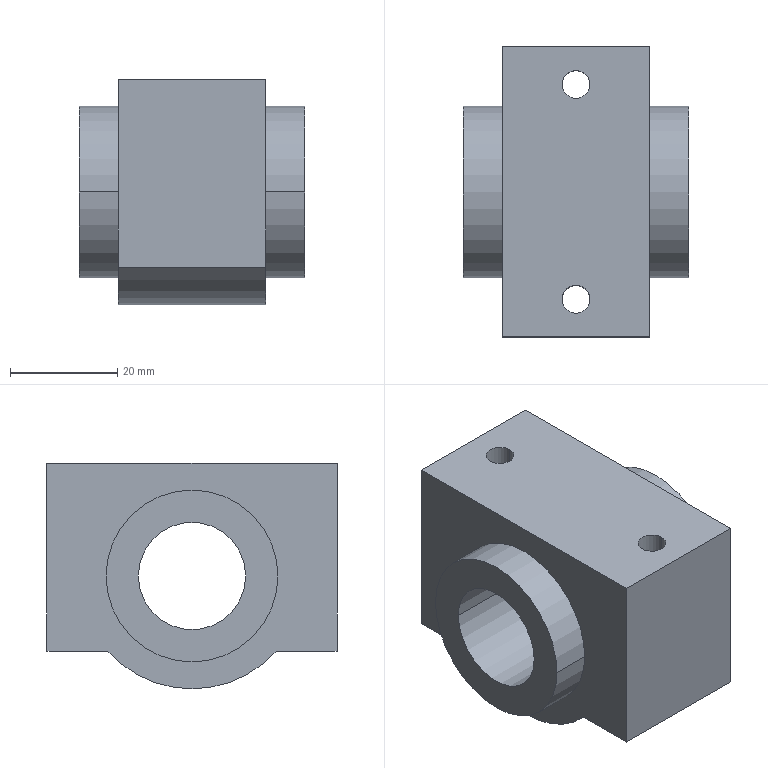Component | SolidWorks | BoxShortLinearBearing-SC20VUU-WERB-2 | 1 solid | 20 faces | box 42 x 54 x 42 mm | volume 53005 mm3 | cylinder 11 | plane 9 | commonest cylinder face diameters 5.2 x4 32 x4 20 x2 42 x1
build123d program:
from build123d import *

# Parameters (mm, degrees)
SKETCH1_R             = 16
SKETCH1_R_2           = 10
EXTRUDE1_DEPTH        = 42
EXTRUDE2_DEPTH        = 13.7
EXTRUDE2_DEPTH_BACK   = 13.7
SKETCH2_R             = 16
M6_TAPPED_HOLE1_D     = 5
M6_TAPPED_HOLE1_DEPTH = 17
M6_TAPPED_HOLE1_TIP   = 1.502
SKETCH5_R             = 2.6
CUT_EXTRUDE1_DEPTH    = 66.246


with BuildPart() as part:
    # Sketch1 → Extrude1 (new body)
    with BuildSketch(Plane.XY):
        with Locations(Location((0, 0, 0), (0, 0, 180))):
            Circle(SKETCH1_R)
        with Locations(Location((0, 0, 0), (0, 0, 180))):
            Circle(SKETCH1_R_2, mode=Mode.SUBTRACT)
    extrude(amount=EXTRUDE1_DEPTH)

    # Sketch2 → Extrude2 (add, two sides: drawn at the far end of the back side and taken through both)
    with BuildSketch(Plane.XY.offset(21).offset(-EXTRUDE2_DEPTH_BACK)):
        with BuildLine():
            Line((15.652, -14), (27, -14))
            Line((27, -14), (27, 21))
            Line((27, 21), (-27, 21))
            Line((-27, 21), (-27, -14))
            Line((-27, -14), (-15.652, -14))
            ThreePointArc((-15.652, -14), (0, -21), (15.652, -14))
        make_face()
        with Locations(Location((0, 0, 0), (0, 0, 180))):
            Circle(SKETCH2_R, mode=Mode.SUBTRACT)
    extrude(amount=EXTRUDE2_DEPTH + EXTRUDE2_DEPTH_BACK)

    # M6 Tapped Hole1
    with Locations(Plane(origin=(0, 21, 0), x_dir=(-1, 0, 0), z_dir=(0, 1, 0))):
        with Locations((20, 21), (-20, 21)):
            Hole(M6_TAPPED_HOLE1_D / 2, depth=M6_TAPPED_HOLE1_DEPTH)
            with Locations((0, 0, -(M6_TAPPED_HOLE1_DEPTH + M6_TAPPED_HOLE1_TIP / 2))):  # 118° drill point
                Cone(0, M6_TAPPED_HOLE1_D / 2, M6_TAPPED_HOLE1_TIP, mode=Mode.SUBTRACT)

    # Sketch5 → Cut-Extrude1 (cut, through all)
    with BuildSketch(Plane(origin=(0, 21, 0), x_dir=(-1, 0, 0), z_dir=(0, 1, 0))):
        with Locations(Location((20, 21, 0), (0, 0, 90))):
            Circle(SKETCH5_R)
        with Locations(Location((-20, 21, 0), (0, 0, 90))):
            Circle(SKETCH5_R)
    extrude(amount=-CUT_EXTRUDE1_DEPTH, mode=Mode.SUBTRACT)


solid = part.part

# Placed as in the assembly
solid = solid.moved(Location((-11.307, 55.443, -26), (90, -90, 0)))
STEP:
#1=COLOUR_RGB('',0.7922,0.8196,0.9333);
#2=FILL_AREA_STYLE_COLOUR('',#1);
#3=FILL_AREA_STYLE('',(#2));
#4=SURFACE_STYLE_FILL_AREA(#3);
#5=SURFACE_SIDE_STYLE('',(#4));
#6=SURFACE_STYLE_USAGE(.BOTH.,#5);
#7=PRESENTATION_STYLE_ASSIGNMENT((#6));
#8=CARTESIAN_POINT('',(-1.17,1.395,-1.575));
#9=VERTEX_POINT('',#8);
#10=CARTESIAN_POINT('',(-1.374,1.395,-1.575));
#11=VERTEX_POINT('',#10);
#12=CARTESIAN_POINT('',(-1.272,1.395,-1.575));
#13=DIRECTION('',(0.,-0.,1.));
#14=DIRECTION('',(-1.,0.,0.));
#15=AXIS2_PLACEMENT_3D('',#12,#13,#14);
#16=CIRCLE('',#15,0.1024);
#17=EDGE_CURVE('',#9,#11,#16,.T.);
#18=ORIENTED_EDGE('',*,*,#17,.F.);
#19=CARTESIAN_POINT('',(-1.17,1.395,-0.1969));
#20=VERTEX_POINT('',#19);
#21=CARTESIAN_POINT('',(-1.17,1.395,-1.85));
#22=DIRECTION('',(0.,-0.,1.));
#23=VECTOR('',#22,39.37);
#24=LINE('',#21,#23);
#25=EDGE_CURVE('',#9,#20,#24,.T.);
#26=ORIENTED_EDGE('',*,*,#25,.T.);
#27=CARTESIAN_POINT('',(-1.374,1.395,-0.1969));
#28=VERTEX_POINT('',#27);
#29=CARTESIAN_POINT('',(-1.272,1.395,-0.1969));
#30=DIRECTION('',(0.,-0.,1.));
#31=DIRECTION('',(-1.,0.,0.));
#32=AXIS2_PLACEMENT_3D('',#29,#30,#31);
#33=CIRCLE('',#32,0.1024);
#34=EDGE_CURVE('',#20,#28,#33,.T.);
#35=ORIENTED_EDGE('',*,*,#34,.T.);
#36=CARTESIAN_POINT('',(-1.374,1.395,-1.85));
#37=DIRECTION('',(0.,-0.,1.));
#38=VECTOR('',#37,39.37);
#39=LINE('',#36,#38);
#40=EDGE_CURVE('',#11,#28,#39,.T.);
#41=ORIENTED_EDGE('',*,*,#40,.F.);
#42=EDGE_LOOP('',(#18,#26,#35,#41));
#43=FACE_OUTER_BOUND('',#42,.T.);
#44=CARTESIAN_POINT('',(-1.272,1.395,-1.85));
#45=DIRECTION('',(0.,-0.,1.));
#46=DIRECTION('',(-1.,0.,0.));
#47=AXIS2_PLACEMENT_3D('',#44,#45,#46);
#48=CYLINDRICAL_SURFACE('',#47,0.1024);
#49=ADVANCED_FACE('',(#43),#48,.F.);
#50=CARTESIAN_POINT('',(-1.17,2.97,-1.575));
#51=VERTEX_POINT('',#50);
#52=CARTESIAN_POINT('',(-1.374,2.97,-1.575));
#53=VERTEX_POINT('',#52);
#54=CARTESIAN_POINT('',(-1.272,2.97,-1.575));
#55=DIRECTION('',(0.,-0.,1.));
#56=DIRECTION('',(-1.,0.,0.));
#57=AXIS2_PLACEMENT_3D('',#54,#55,#56);
#58=CIRCLE('',#57,0.1024);
#59=EDGE_CURVE('',#51,#53,#58,.T.);
#60=ORIENTED_EDGE('',*,*,#59,.F.);
#61=CARTESIAN_POINT('',(-1.17,2.97,-0.1969));
#62=VERTEX_POINT('',#61);
#63=CARTESIAN_POINT('',(-1.17,2.97,-1.85));
#64=DIRECTION('',(0.,-0.,1.));
#65=VECTOR('',#64,39.37);
#66=LINE('',#63,#65);
#67=EDGE_CURVE('',#51,#62,#66,.T.);
#68=ORIENTED_EDGE('',*,*,#67,.T.);
#69=CARTESIAN_POINT('',(-1.374,2.97,-0.1969));
#70=VERTEX_POINT('',#69);
#71=CARTESIAN_POINT('',(-1.272,2.97,-0.1969));
#72=DIRECTION('',(0.,-0.,1.));
#73=DIRECTION('',(-1.,0.,0.));
#74=AXIS2_PLACEMENT_3D('',#71,#72,#73);
#75=CIRCLE('',#74,0.1024);
#76=EDGE_CURVE('',#62,#70,#75,.T.);
#77=ORIENTED_EDGE('',*,*,#76,.T.);
#78=CARTESIAN_POINT('',(-1.374,2.97,-1.85));
#79=DIRECTION('',(0.,-0.,1.));
#80=VECTOR('',#79,39.37);
#81=LINE('',#78,#80);
#82=EDGE_CURVE('',#53,#70,#81,.T.);
#83=ORIENTED_EDGE('',*,*,#82,.F.);
#84=EDGE_LOOP('',(#60,#68,#77,#83));
#85=FACE_OUTER_BOUND('',#84,.T.);
#86=CARTESIAN_POINT('',(-1.272,2.97,-1.85));
#87=DIRECTION('',(0.,-0.,1.));
#88=DIRECTION('',(-1.,0.,0.));
#89=AXIS2_PLACEMENT_3D('',#86,#87,#88);
#90=CYLINDRICAL_SURFACE('',#89,0.1024);
#91=ADVANCED_FACE('',(#85),#90,.F.);
#92=CARTESIAN_POINT('',(-2.099,2.576,-1.024));
#93=VERTEX_POINT('',#92);
#94=CARTESIAN_POINT('',(-2.099,1.789,-1.024));
#95=VERTEX_POINT('',#94);
#96=CARTESIAN_POINT('',(-2.099,2.183,-1.024));
#97=DIRECTION('',(-1.,-0.,0.));
#98=DIRECTION('',(0.,-1.,0.));
#99=AXIS2_PLACEMENT_3D('',#96,#97,#98);
#100=CIRCLE('',#99,0.3937);
#101=EDGE_CURVE('',#93,#95,#100,.T.);
#102=ORIENTED_EDGE('',*,*,#101,.T.);
#103=CARTESIAN_POINT('',(-0.4452,1.789,-1.024));
#104=VERTEX_POINT('',#103);
#105=CARTESIAN_POINT('',(-2.099,1.789,-1.024));
#106=DIRECTION('',(1.,0.,-0.));
#107=VECTOR('',#106,39.37);
#108=LINE('',#105,#107);
#109=EDGE_CURVE('',#95,#104,#108,.T.);
#110=ORIENTED_EDGE('',*,*,#109,.T.);
#111=CARTESIAN_POINT('',(-0.4452,2.576,-1.024));
#112=VERTEX_POINT('',#111);
#113=CARTESIAN_POINT('',(-0.4452,2.183,-1.024));
#114=DIRECTION('',(-1.,-0.,0.));
#115=DIRECTION('',(0.,-1.,0.));
#116=AXIS2_PLACEMENT_3D('',#113,#114,#115);
#117=CIRCLE('',#116,0.3937);
#118=EDGE_CURVE('',#112,#104,#117,.T.);
#119=ORIENTED_EDGE('',*,*,#118,.F.);
#120=CARTESIAN_POINT('',(-2.099,2.576,-1.024));
#121=DIRECTION('',(1.,0.,-0.));
#122=VECTOR('',#121,39.37);
#123=LINE('',#120,#122);
#124=EDGE_CURVE('',#93,#112,#123,.T.);
#125=ORIENTED_EDGE('',*,*,#124,.F.);
#126=EDGE_LOOP('',(#102,#110,#119,#125));
#127=FACE_OUTER_BOUND('',#126,.T.);
#128=CARTESIAN_POINT('',(-2.099,2.183,-1.024));
#129=DIRECTION('',(1.,0.,-0.));
#130=DIRECTION('',(0.,1.,0.));
#131=AXIS2_PLACEMENT_3D('',#128,#129,#130);
#132=CYLINDRICAL_SURFACE('',#131,0.3937);
#133=ADVANCED_FACE('',(#127),#132,.F.);
#134=CARTESIAN_POINT('',(-2.099,1.553,-1.024));
#135=VERTEX_POINT('',#134);
#136=CARTESIAN_POINT('',(-2.099,2.813,-1.024));
#137=VERTEX_POINT('',#136);
#138=CARTESIAN_POINT('',(-2.099,2.183,-1.024));
#139=DIRECTION('',(-1.,-0.,0.));
#140=DIRECTION('',(0.,-1.,0.));
#141=AXIS2_PLACEMENT_3D('',#138,#139,#140);
#142=CIRCLE('',#141,0.6299);
#143=EDGE_CURVE('',#135,#137,#142,.T.);
#144=ORIENTED_EDGE('',*,*,#143,.F.);
#145=CARTESIAN_POINT('',(-1.811,1.553,-1.024));
#146=VERTEX_POINT('',#145);
#147=CARTESIAN_POINT('',(-2.099,1.553,-1.024));
#148=DIRECTION('',(1.,0.,-0.));
#149=VECTOR('',#148,39.37);
#150=LINE('',#147,#149);
#151=EDGE_CURVE('',#135,#146,#150,.T.);
#152=ORIENTED_EDGE('',*,*,#151,.T.);
#153=CARTESIAN_POINT('',(-1.811,2.813,-1.024));
#154=VERTEX_POINT('',#153);
#155=CARTESIAN_POINT('',(-1.811,2.183,-1.024));
#156=DIRECTION('',(-1.,-0.,0.));
#157=DIRECTION('',(0.,-1.,0.));
#158=AXIS2_PLACEMENT_3D('',#155,#156,#157);
#159=CIRCLE('',#158,0.6299);
#160=EDGE_CURVE('',#146,#154,#159,.T.);
#161=ORIENTED_EDGE('',*,*,#160,.T.);
#162=CARTESIAN_POINT('',(-2.099,2.813,-1.024));
#163=DIRECTION('',(1.,0.,-0.));
#164=VECTOR('',#163,39.37);
#165=LINE('',#162,#164);
#166=EDGE_CURVE('',#137,#154,#165,.T.);
#167=ORIENTED_EDGE('',*,*,#166,.F.);
#168=EDGE_LOOP('',(#144,#152,#161,#167));
#169=FACE_OUTER_BOUND('',#168,.T.);
#170=CARTESIAN_POINT('',(-2.099,2.183,-1.024));
#171=DIRECTION('',(1.,0.,-0.));
#172=DIRECTION('',(0.,1.,0.));
#173=AXIS2_PLACEMENT_3D('',#170,#171,#172);
#174=CYLINDRICAL_SURFACE('',#173,0.6299);
#175=ADVANCED_FACE('',(#169),#174,.T.);
#176=CARTESIAN_POINT('',(-0.7326,1.553,-1.024));
#177=VERTEX_POINT('',#176);
#178=CARTESIAN_POINT('',(-0.7326,2.813,-1.024));
#179=VERTEX_POINT('',#178);
#180=CARTESIAN_POINT('',(-0.7326,2.183,-1.024));
#181=DIRECTION('',(-1.,-0.,0.));
#182=DIRECTION('',(0.,-1.,0.));
#183=AXIS2_PLACEMENT_3D('',#180,#181,#182);
#184=CIRCLE('',#183,0.6299);
#185=EDGE_CURVE('',#177,#179,#184,.T.);
#186=ORIENTED_EDGE('',*,*,#185,.F.);
#187=CARTESIAN_POINT('',(-0.4452,1.553,-1.024));
#188=VERTEX_POINT('',#187);
#189=CARTESIAN_POINT('',(-2.099,1.553,-1.024));
#190=DIRECTION('',(1.,0.,-0.));
#191=VECTOR('',#190,39.37);
#192=LINE('',#189,#191);
#193=EDGE_CURVE('',#177,#188,#192,.T.);
#194=ORIENTED_EDGE('',*,*,#193,.T.);
#195=CARTESIAN_POINT('',(-0.4452,2.813,-1.024));
#196=VERTEX_POINT('',#195);
#197=CARTESIAN_POINT('',(-0.4452,2.183,-1.024));
#198=DIRECTION('',(-1.,-0.,0.));
#199=DIRECTION('',(0.,-1.,0.));
#200=AXIS2_PLACEMENT_3D('',#197,#198,#199);
#201=CIRCLE('',#200,0.6299);
#202=EDGE_CURVE('',#188,#196,#201,.T.);
#203=ORIENTED_EDGE('',*,*,#202,.T.);
#204=CARTESIAN_POINT('',(-2.099,2.813,-1.024));
#205=DIRECTION('',(1.,0.,-0.));
#206=VECTOR('',#205,39.37);
#207=LINE('',#204,#206);
#208=EDGE_CURVE('',#179,#196,#207,.T.);
#209=ORIENTED_EDGE('',*,*,#208,.F.);
#210=EDGE_LOOP('',(#186,#194,#203,#209));
#211=FACE_OUTER_BOUND('',#210,.T.);
#212=CARTESIAN_POINT('',(-2.099,2.183,-1.024));
#213=DIRECTION('',(1.,0.,-0.));
#214=DIRECTION('',(0.,1.,0.));
#215=AXIS2_PLACEMENT_3D('',#212,#213,#214);
#216=CYLINDRICAL_SURFACE('',#215,0.6299);
#217=ADVANCED_FACE('',(#211),#216,.T.);
#218=ORIENTED_EDGE('',*,*,#193,.F.);
#219=CARTESIAN_POINT('',(-0.7326,2.183,-1.024));
#220=DIRECTION('',(-1.,-0.,0.));
#221=DIRECTION('',(0.,-1.,0.));
#222=AXIS2_PLACEMENT_3D('',#219,#220,#221);
#223=CIRCLE('',#222,0.6299);
#224=EDGE_CURVE('',#179,#177,#223,.T.);
#225=ORIENTED_EDGE('',*,*,#224,.F.);
#226=ORIENTED_EDGE('',*,*,#208,.T.);
#227=CARTESIAN_POINT('',(-0.4452,2.183,-1.024));
#228=DIRECTION('',(-1.,-0.,0.));
#229=DIRECTION('',(0.,-1.,0.));
#230=AXIS2_PLACEMENT_3D('',#227,#228,#229);
#231=CIRCLE('',#230,0.6299);
#232=EDGE_CURVE('',#196,#188,#231,.T.);
#233=ORIENTED_EDGE('',*,*,#232,.T.);
#234=EDGE_LOOP('',(#218,#225,#226,#233));
#235=FACE_OUTER_BOUND('',#234,.T.);
#236=CARTESIAN_POINT('',(-2.099,2.183,-1.024));
#237=DIRECTION('',(1.,0.,-0.));
#238=DIRECTION('',(0.,1.,0.));
#239=AXIS2_PLACEMENT_3D('',#236,#237,#238);
#240=CYLINDRICAL_SURFACE('',#239,0.6299);
#241=ADVANCED_FACE('',(#235),#240,.T.);
#242=CARTESIAN_POINT('',(-2.099,2.183,-1.024));
#243=DIRECTION('',(-1.,-0.,0.));
#244=DIRECTION('',(0.,-1.,0.));
#245=AXIS2_PLACEMENT_3D('',#242,#243,#244);
#246=CIRCLE('',#245,0.6299);
#247=EDGE_CURVE('',#137,#135,#246,.T.);
#248=ORIENTED_EDGE('',*,*,#247,.T.);
#249=ORIENTED_EDGE('',*,*,#143,.T.);
#250=EDGE_LOOP('',(#248,#249));
#251=FACE_OUTER_BOUND('',#250,.T.);
#252=ORIENTED_EDGE('',*,*,#101,.F.);
#253=CARTESIAN_POINT('',(-2.099,2.183,-1.024));
#254=DIRECTION('',(-1.,-0.,0.));
#255=DIRECTION('',(0.,-1.,0.));
#256=AXIS2_PLACEMENT_3D('',#253,#254,#255);
#257=CIRCLE('',#256,0.3937);
#258=EDGE_CURVE('',#95,#93,#257,.T.);
#259=ORIENTED_EDGE('',*,*,#258,.F.);
#260=EDGE_LOOP('',(#252,#259));
#261=FACE_BOUND('',#260,.T.);
#262=CARTESIAN_POINT('',(-2.099,2.183,-1.024));
#263=DIRECTION('',(-1.,0.,0.));
#264=DIRECTION('',(-0.,-1.,0.));
#265=AXIS2_PLACEMENT_3D('',#262,#263,#264);
#266=PLANE('',#265);
#267=ADVANCED_FACE('',(#251,#261),#266,.T.);
#268=ORIENTED_EDGE('',*,*,#232,.F.);
#269=ORIENTED_EDGE('',*,*,#202,.F.);
#270=EDGE_LOOP('',(#268,#269));
#271=FACE_OUTER_BOUND('',#270,.T.);
#272=ORIENTED_EDGE('',*,*,#118,.T.);
#273=CARTESIAN_POINT('',(-0.4452,2.183,-1.024));
#274=DIRECTION('',(-1.,-0.,0.));
#275=DIRECTION('',(0.,-1.,0.));
#276=AXIS2_PLACEMENT_3D('',#273,#274,#275);
#277=CIRCLE('',#276,0.3937);
#278=EDGE_CURVE('',#104,#112,#277,.T.);
#279=ORIENTED_EDGE('',*,*,#278,.T.);
#280=EDGE_LOOP('',(#272,#279));
#281=FACE_BOUND('',#280,.T.);
#282=CARTESIAN_POINT('',(-0.4452,2.183,-1.024));
#283=DIRECTION('',(-1.,0.,0.));
#284=DIRECTION('',(-0.,-1.,0.));
#285=AXIS2_PLACEMENT_3D('',#282,#283,#284);
#286=PLANE('',#285);
#287=ADVANCED_FACE('',(#271,#281),#286,.F.);
#288=ORIENTED_EDGE('',*,*,#151,.F.);
#289=ORIENTED_EDGE('',*,*,#247,.F.);
#290=ORIENTED_EDGE('',*,*,#166,.T.);
#291=CARTESIAN_POINT('',(-1.811,2.183,-1.024));
#292=DIRECTION('',(-1.,-0.,0.));
#293=DIRECTION('',(0.,-1.,0.));
#294=AXIS2_PLACEMENT_3D('',#291,#292,#293);
#295=CIRCLE('',#294,0.6299);
#296=EDGE_CURVE('',#154,#146,#295,.T.);
#297=ORIENTED_EDGE('',*,*,#296,.T.);
#298=EDGE_LOOP('',(#288,#289,#290,#297));
#299=FACE_OUTER_BOUND('',#298,.T.);
#300=CARTESIAN_POINT('',(-2.099,2.183,-1.024));
#301=DIRECTION('',(1.,0.,-0.));
#302=DIRECTION('',(0.,1.,0.));
#303=AXIS2_PLACEMENT_3D('',#300,#301,#302);
#304=CYLINDRICAL_SURFACE('',#303,0.6299);
#305=ADVANCED_FACE('',(#299),#304,.T.);
#306=ORIENTED_EDGE('',*,*,#109,.F.);
#307=ORIENTED_EDGE('',*,*,#258,.T.);
#308=ORIENTED_EDGE('',*,*,#124,.T.);
#309=ORIENTED_EDGE('',*,*,#278,.F.);
#310=EDGE_LOOP('',(#306,#307,#308,#309));
#311=FACE_OUTER_BOUND('',#310,.T.);
#312=CARTESIAN_POINT('',(-2.099,2.183,-1.024));
#313=DIRECTION('',(1.,0.,-0.));
#314=DIRECTION('',(0.,1.,0.));
#315=AXIS2_PLACEMENT_3D('',#312,#313,#314);
#316=CYLINDRICAL_SURFACE('',#315,0.3937);
#317=ADVANCED_FACE('',(#311),#316,.F.);
#318=CARTESIAN_POINT('',(-1.811,3.246,-0.1969));
#319=VERTEX_POINT('',#318);
#320=CARTESIAN_POINT('',(-1.811,3.246,-1.575));
#321=VERTEX_POINT('',#320);
#322=CARTESIAN_POINT('',(-1.811,3.246,-0.1969));
#323=DIRECTION('',(-0.,0.,-1.));
#324=VECTOR('',#323,39.37);
#325=LINE('',#322,#324);
#326=EDGE_CURVE('',#319,#321,#325,.T.);
#327=ORIENTED_EDGE('',*,*,#326,.T.);
#328=CARTESIAN_POINT('',(-1.811,2.799,-1.575));
#329=VERTEX_POINT('',#328);
#330=CARTESIAN_POINT('',(-1.811,3.246,-1.575));
#331=DIRECTION('',(-0.,-1.,0.));
#332=VECTOR('',#331,39.37);
#333=LINE('',#330,#332);
#334=EDGE_CURVE('',#321,#329,#333,.T.);
#335=ORIENTED_EDGE('',*,*,#334,.T.);
#336=CARTESIAN_POINT('',(-1.811,1.567,-1.575));
#337=VERTEX_POINT('',#336);
#338=CARTESIAN_POINT('',(-1.811,2.183,-1.024));
#339=DIRECTION('',(-1.,-0.,0.));
#340=DIRECTION('',(0.,-1.,0.));
#341=AXIS2_PLACEMENT_3D('',#338,#339,#340);
#342=CIRCLE('',#341,0.8268);
#343=EDGE_CURVE('',#329,#337,#342,.T.);
#344=ORIENTED_EDGE('',*,*,#343,.T.);
#345=CARTESIAN_POINT('',(-1.811,1.12,-1.575));
#346=VERTEX_POINT('',#345);
#347=CARTESIAN_POINT('',(-1.811,1.567,-1.575));
#348=DIRECTION('',(-0.,-1.,0.));
#349=VECTOR('',#348,39.37);
#350=LINE('',#347,#349);
#351=EDGE_CURVE('',#337,#346,#350,.T.);
#352=ORIENTED_EDGE('',*,*,#351,.T.);
#353=CARTESIAN_POINT('',(-1.811,1.12,-0.1969));
#354=VERTEX_POINT('',#353);
#355=CARTESIAN_POINT('',(-1.811,1.12,-0.1969));
#356=DIRECTION('',(0.,-0.,1.));
#357=VECTOR('',#356,39.37);
#358=LINE('',#355,#357);
#359=EDGE_CURVE('',#346,#354,#358,.T.);
#360=ORIENTED_EDGE('',*,*,#359,.T.);
#361=CARTESIAN_POINT('',(-1.811,3.246,-0.1969));
#362=DIRECTION('',(0.,1.,-0.));
#363=VECTOR('',#362,39.37);
#364=LINE('',#361,#363);
#365=EDGE_CURVE('',#354,#319,#364,.T.);
#366=ORIENTED_EDGE('',*,*,#365,.T.);
#367=EDGE_LOOP('',(#327,#335,#344,#352,#360,#366));
#368=FACE_OUTER_BOUND('',#367,.T.);
#369=ORIENTED_EDGE('',*,*,#296,.F.);
#370=ORIENTED_EDGE('',*,*,#160,.F.);
#371=EDGE_LOOP('',(#369,#370));
#372=FACE_BOUND('',#371,.T.);
#373=CARTESIAN_POINT('',(-1.811,2.183,-1.024));
#374=DIRECTION('',(-1.,0.,0.));
#375=DIRECTION('',(-0.,-1.,0.));
#376=AXIS2_PLACEMENT_3D('',#373,#374,#375);
#377=PLANE('',#376);
#378=ADVANCED_FACE('',(#368,#372),#377,.T.);
#379=CARTESIAN_POINT('',(-0.7326,3.246,-0.1969));
#380=VERTEX_POINT('',#379);
#381=CARTESIAN_POINT('',(-1.811,3.246,-0.1969));
#382=DIRECTION('',(1.,0.,-0.));
#383=VECTOR('',#382,39.37);
#384=LINE('',#381,#383);
#385=EDGE_CURVE('',#319,#380,#384,.T.);
#386=ORIENTED_EDGE('',*,*,#385,.T.);
#387=CARTESIAN_POINT('',(-0.7326,3.246,-1.575));
#388=VERTEX_POINT('',#387);
#389=CARTESIAN_POINT('',(-0.7326,3.246,-0.1969));
#390=DIRECTION('',(-0.,0.,-1.));
#391=VECTOR('',#390,39.37);
#392=LINE('',#389,#391);
#393=EDGE_CURVE('',#380,#388,#392,.T.);
#394=ORIENTED_EDGE('',*,*,#393,.T.);
#395=CARTESIAN_POINT('',(-1.811,3.246,-1.575));
#396=DIRECTION('',(1.,0.,-0.));
#397=VECTOR('',#396,39.37);
#398=LINE('',#395,#397);
#399=EDGE_CURVE('',#321,#388,#398,.T.);
#400=ORIENTED_EDGE('',*,*,#399,.F.);
#401=ORIENTED_EDGE('',*,*,#326,.F.);
#402=EDGE_LOOP('',(#386,#394,#400,#401));
#403=FACE_OUTER_BOUND('',#402,.T.);
#404=CARTESIAN_POINT('',(-1.811,3.246,-0.1969));
#405=DIRECTION('',(0.,-1.,0.));
#406=DIRECTION('',(1.,0.,-0.));
#407=AXIS2_PLACEMENT_3D('',#404,#405,#406);
#408=PLANE('',#407);
#409=ADVANCED_FACE('',(#403),#408,.F.);
#410=CARTESIAN_POINT('',(-1.272,2.97,-1.575));
#411=DIRECTION('',(0.,-0.,1.));
#412=DIRECTION('',(-1.,0.,0.));
#413=AXIS2_PLACEMENT_3D('',#410,#411,#412);
#414=CIRCLE('',#413,0.1024);
#415=EDGE_CURVE('',#53,#51,#414,.T.);
#416=ORIENTED_EDGE('',*,*,#415,.T.);
#417=ORIENTED_EDGE('',*,*,#59,.T.);
#418=EDGE_LOOP('',(#416,#417));
#419=FACE_BOUND('',#418,.T.);
#420=ORIENTED_EDGE('',*,*,#399,.T.);
#421=CARTESIAN_POINT('',(-0.7326,2.799,-1.575));
#422=VERTEX_POINT('',#421);
#423=CARTESIAN_POINT('',(-0.7326,3.246,-1.575));
#424=DIRECTION('',(-0.,-1.,0.));
#425=VECTOR('',#424,39.37);
#426=LINE('',#423,#425);
#427=EDGE_CURVE('',#388,#422,#426,.T.);
#428=ORIENTED_EDGE('',*,*,#427,.T.);
#429=CARTESIAN_POINT('',(-1.811,2.799,-1.575));
#430=DIRECTION('',(1.,0.,-0.));
#431=VECTOR('',#430,39.37);
#432=LINE('',#429,#431);
#433=EDGE_CURVE('',#329,#422,#432,.T.);
#434=ORIENTED_EDGE('',*,*,#433,.F.);
#435=ORIENTED_EDGE('',*,*,#334,.F.);
#436=EDGE_LOOP('',(#420,#428,#434,#435));
#437=FACE_OUTER_BOUND('',#436,.T.);
#438=CARTESIAN_POINT('',(-1.811,3.246,-1.575));
#439=DIRECTION('',(0.,-0.,1.));
#440=DIRECTION('',(-1.,-0.,0.));
#441=AXIS2_PLACEMENT_3D('',#438,#439,#440);
#442=PLANE('',#441);
#443=ADVANCED_FACE('',(#419,#437),#442,.F.);
#444=ORIENTED_EDGE('',*,*,#433,.T.);
#445=CARTESIAN_POINT('',(-0.7326,1.567,-1.575));
#446=VERTEX_POINT('',#445);
#447=CARTESIAN_POINT('',(-0.7326,2.183,-1.024));
#448=DIRECTION('',(-1.,-0.,0.));
#449=DIRECTION('',(0.,-1.,0.));
#450=AXIS2_PLACEMENT_3D('',#447,#448,#449);
#451=CIRCLE('',#450,0.8268);
#452=EDGE_CURVE('',#422,#446,#451,.T.);
#453=ORIENTED_EDGE('',*,*,#452,.T.);
#454=CARTESIAN_POINT('',(-1.811,1.567,-1.575));
#455=DIRECTION('',(1.,0.,-0.));
#456=VECTOR('',#455,39.37);
#457=LINE('',#454,#456);
#458=EDGE_CURVE('',#337,#446,#457,.T.);
#459=ORIENTED_EDGE('',*,*,#458,.F.);
#460=ORIENTED_EDGE('',*,*,#343,.F.);
#461=EDGE_LOOP('',(#444,#453,#459,#460));
#462=FACE_OUTER_BOUND('',#461,.T.);
#463=CARTESIAN_POINT('',(-1.811,2.183,-1.024));
#464=DIRECTION('',(1.,0.,-0.));
#465=DIRECTION('',(0.,1.,0.));
#466=AXIS2_PLACEMENT_3D('',#463,#464,#465);
#467=CYLINDRICAL_SURFACE('',#466,0.8268);
#468=ADVANCED_FACE('',(#462),#467,.T.);
#469=CARTESIAN_POINT('',(-1.272,1.395,-1.575));
#470=DIRECTION('',(0.,-0.,1.));
#471=DIRECTION('',(-1.,0.,0.));
#472=AXIS2_PLACEMENT_3D('',#469,#470,#471);
#473=CIRCLE('',#472,0.1024);
#474=EDGE_CURVE('',#11,#9,#473,.T.);
#475=ORIENTED_EDGE('',*,*,#474,.T.);
#476=ORIENTED_EDGE('',*,*,#17,.T.);
#477=EDGE_LOOP('',(#475,#476));
#478=FACE_BOUND('',#477,.T.);
#479=ORIENTED_EDGE('',*,*,#458,.T.);
#480=CARTESIAN_POINT('',(-0.7326,1.12,-1.575));
#481=VERTEX_POINT('',#480);
#482=CARTESIAN_POINT('',(-0.7326,1.567,-1.575));
#483=DIRECTION('',(-0.,-1.,0.));
#484=VECTOR('',#483,39.37);
#485=LINE('',#482,#484);
#486=EDGE_CURVE('',#446,#481,#485,.T.);
#487=ORIENTED_EDGE('',*,*,#486,.T.);
#488=CARTESIAN_POINT('',(-1.811,1.12,-1.575));
#489=DIRECTION('',(1.,0.,-0.));
#490=VECTOR('',#489,39.37);
#491=LINE('',#488,#490);
#492=EDGE_CURVE('',#346,#481,#491,.T.);
#493=ORIENTED_EDGE('',*,*,#492,.F.);
#494=ORIENTED_EDGE('',*,*,#351,.F.);
#495=EDGE_LOOP('',(#479,#487,#493,#494));
#496=FACE_OUTER_BOUND('',#495,.T.);
#497=CARTESIAN_POINT('',(-1.811,1.567,-1.575));
#498=DIRECTION('',(0.,-0.,1.));
#499=DIRECTION('',(-1.,-0.,0.));
#500=AXIS2_PLACEMENT_3D('',#497,#498,#499);
#501=PLANE('',#500);
#502=ADVANCED_FACE('',(#478,#496),#501,.F.);
#503=ORIENTED_EDGE('',*,*,#492,.T.);
#504=CARTESIAN_POINT('',(-0.7326,1.12,-0.1969));
#505=VERTEX_POINT('',#504);
#506=CARTESIAN_POINT('',(-0.7326,1.12,-0.1969));
#507=DIRECTION('',(0.,-0.,1.));
#508=VECTOR('',#507,39.37);
#509=LINE('',#506,#508);
#510=EDGE_CURVE('',#481,#505,#509,.T.);
#511=ORIENTED_EDGE('',*,*,#510,.T.);
#512=CARTESIAN_POINT('',(-1.811,1.12,-0.1969));
#513=DIRECTION('',(1.,0.,-0.));
#514=VECTOR('',#513,39.37);
#515=LINE('',#512,#514);
#516=EDGE_CURVE('',#354,#505,#515,.T.);
#517=ORIENTED_EDGE('',*,*,#516,.F.);
#518=ORIENTED_EDGE('',*,*,#359,.F.);
#519=EDGE_LOOP('',(#503,#511,#517,#518));
#520=FACE_OUTER_BOUND('',#519,.T.);
#521=CARTESIAN_POINT('',(-1.811,1.12,-0.1969));
#522=DIRECTION('',(0.,1.,0.));
#523=DIRECTION('',(-0.,0.,-1.));
#524=AXIS2_PLACEMENT_3D('',#521,#522,#523);
#525=PLANE('',#524);
#526=ADVANCED_FACE('',(#520),#525,.F.);
#527=CARTESIAN_POINT('',(-1.272,1.395,-0.1969));
#528=DIRECTION('',(0.,-0.,1.));
#529=DIRECTION('',(-1.,0.,0.));
#530=AXIS2_PLACEMENT_3D('',#527,#528,#529);
#531=CIRCLE('',#530,0.1024);
#532=EDGE_CURVE('',#28,#20,#531,.T.);
#533=ORIENTED_EDGE('',*,*,#532,.F.);
#534=ORIENTED_EDGE('',*,*,#34,.F.);
#535=EDGE_LOOP('',(#533,#534));
#536=FACE_BOUND('',#535,.T.);
#537=CARTESIAN_POINT('',(-1.272,2.97,-0.1969));
#538=DIRECTION('',(0.,-0.,1.));
#539=DIRECTION('',(-1.,0.,0.));
#540=AXIS2_PLACEMENT_3D('',#537,#538,#539);
#541=CIRCLE('',#540,0.1024);
#542=EDGE_CURVE('',#70,#62,#541,.T.);
#543=ORIENTED_EDGE('',*,*,#542,.F.);
#544=ORIENTED_EDGE('',*,*,#76,.F.);
#545=EDGE_LOOP('',(#543,#544));
#546=FACE_BOUND('',#545,.T.);
#547=ORIENTED_EDGE('',*,*,#516,.T.);
#548=CARTESIAN_POINT('',(-0.7326,3.246,-0.1969));
#549=DIRECTION('',(0.,1.,-0.));
#550=VECTOR('',#549,39.37);
#551=LINE('',#548,#550);
#552=EDGE_CURVE('',#505,#380,#551,.T.);
#553=ORIENTED_EDGE('',*,*,#552,.T.);
#554=ORIENTED_EDGE('',*,*,#385,.F.);
#555=ORIENTED_EDGE('',*,*,#365,.F.);
#556=EDGE_LOOP('',(#547,#553,#554,#555));
#557=FACE_OUTER_BOUND('',#556,.T.);
#558=CARTESIAN_POINT('',(-1.811,3.246,-0.1969));
#559=DIRECTION('',(-0.,0.,-1.));
#560=DIRECTION('',(1.,0.,-0.));
#561=AXIS2_PLACEMENT_3D('',#558,#559,#560);
#562=PLANE('',#561);
#563=ADVANCED_FACE('',(#536,#546,#557),#562,.F.);
#564=ORIENTED_EDGE('',*,*,#224,.T.);
#565=ORIENTED_EDGE('',*,*,#185,.T.);
#566=EDGE_LOOP('',(#564,#565));
#567=FACE_BOUND('',#566,.T.);
#568=ORIENTED_EDGE('',*,*,#393,.F.);
#569=ORIENTED_EDGE('',*,*,#552,.F.);
#570=ORIENTED_EDGE('',*,*,#510,.F.);
#571=ORIENTED_EDGE('',*,*,#486,.F.);
#572=ORIENTED_EDGE('',*,*,#452,.F.);
#573=ORIENTED_EDGE('',*,*,#427,.F.);
#574=EDGE_LOOP('',(#568,#569,#570,#571,#572,#573));
#575=FACE_OUTER_BOUND('',#574,.T.);
#576=CARTESIAN_POINT('',(-0.7326,2.183,-1.024));
#577=DIRECTION('',(-1.,0.,0.));
#578=DIRECTION('',(-0.,-1.,0.));
#579=AXIS2_PLACEMENT_3D('',#576,#577,#578);
#580=PLANE('',#579);
#581=ADVANCED_FACE('',(#567,#575),#580,.F.);
#582=ORIENTED_EDGE('',*,*,#67,.F.);
#583=ORIENTED_EDGE('',*,*,#415,.F.);
#584=ORIENTED_EDGE('',*,*,#82,.T.);
#585=ORIENTED_EDGE('',*,*,#542,.T.);
#586=EDGE_LOOP('',(#582,#583,#584,#585));
#587=FACE_OUTER_BOUND('',#586,.T.);
#588=CARTESIAN_POINT('',(-1.272,2.97,-1.85));
#589=DIRECTION('',(0.,-0.,1.));
#590=DIRECTION('',(-1.,0.,0.));
#591=AXIS2_PLACEMENT_3D('',#588,#589,#590);
#592=CYLINDRICAL_SURFACE('',#591,0.1024);
#593=ADVANCED_FACE('',(#587),#592,.F.);
#594=ORIENTED_EDGE('',*,*,#25,.F.);
#595=ORIENTED_EDGE('',*,*,#474,.F.);
#596=ORIENTED_EDGE('',*,*,#40,.T.);
#597=ORIENTED_EDGE('',*,*,#532,.T.);
#598=EDGE_LOOP('',(#594,#595,#596,#597));
#599=FACE_OUTER_BOUND('',#598,.T.);
#600=CARTESIAN_POINT('',(-1.272,1.395,-1.85));
#601=DIRECTION('',(0.,-0.,1.));
#602=DIRECTION('',(-1.,0.,0.));
#603=AXIS2_PLACEMENT_3D('',#600,#601,#602);
#604=CYLINDRICAL_SURFACE('',#603,0.1024);
#605=ADVANCED_FACE('',(#599),#604,.F.);
#606=CLOSED_SHELL('',(#49,#91,#133,#175,#217,#241,#267,#287,#305,#317,#378,#409,#443,#468,#502,#526,#563,#581,#593,#605));
#607=MANIFOLD_SOLID_BREP('',#606);
#608=STYLED_ITEM('',(#7),#607);
#609=(LENGTH_UNIT()NAMED_UNIT(*)SI_UNIT($,.METRE.));
#610=LENGTH_MEASURE_WITH_UNIT(LENGTH_MEASURE(0.0254),#609);
#611=DIMENSIONAL_EXPONENTS(1.,0.,0.,0.,0.,0.,0.);
#612=(CONVERSION_BASED_UNIT('',#610)LENGTH_UNIT()NAMED_UNIT(#611));
#613=UNCERTAINTY_MEASURE_WITH_UNIT(LENGTH_MEASURE(0.00001),#612,'','');
#614=(NAMED_UNIT(*)PLANE_ANGLE_UNIT()SI_UNIT($,.RADIAN.));
#615=(NAMED_UNIT(*)SI_UNIT($,.STERADIAN.)SOLID_ANGLE_UNIT());
#616=(GEOMETRIC_REPRESENTATION_CONTEXT(3)GLOBAL_UNCERTAINTY_ASSIGNED_CONTEXT((#613))GLOBAL_UNIT_ASSIGNED_CONTEXT((#612,#614,#615))REPRESENTATION_CONTEXT('',''));
#617=MECHANICAL_DESIGN_GEOMETRIC_PRESENTATION_REPRESENTATION('',(#608),#616);
#618=CARTESIAN_POINT('',(0.,0.,0.));
#619=DIRECTION('',(0.,0.,1.));
#620=DIRECTION('',(1.,0.,0.));
#621=AXIS2_PLACEMENT_3D('',#618,#619,#620);
#622=(LENGTH_UNIT()NAMED_UNIT(*)SI_UNIT($,.METRE.));
#623=LENGTH_MEASURE_WITH_UNIT(LENGTH_MEASURE(0.0254),#622);
#624=DIMENSIONAL_EXPONENTS(1.,0.,0.,0.,0.,0.,0.);
#625=(CONVERSION_BASED_UNIT('',#623)LENGTH_UNIT()NAMED_UNIT(#624));
#626=UNCERTAINTY_MEASURE_WITH_UNIT(LENGTH_MEASURE(0.00001),#625,'','');
#627=(NAMED_UNIT(*)PLANE_ANGLE_UNIT()SI_UNIT($,.RADIAN.));
#628=(NAMED_UNIT(*)SI_UNIT($,.STERADIAN.)SOLID_ANGLE_UNIT());
#629=(GEOMETRIC_REPRESENTATION_CONTEXT(3)GLOBAL_UNCERTAINTY_ASSIGNED_CONTEXT((#626))GLOBAL_UNIT_ASSIGNED_CONTEXT((#625,#627,#628))REPRESENTATION_CONTEXT('',''));
#630=ADVANCED_BREP_SHAPE_REPRESENTATION('',(#607,#621),#629);
#631=PRESENTATION_LAYER_ASSIGNMENT('','',(#608));